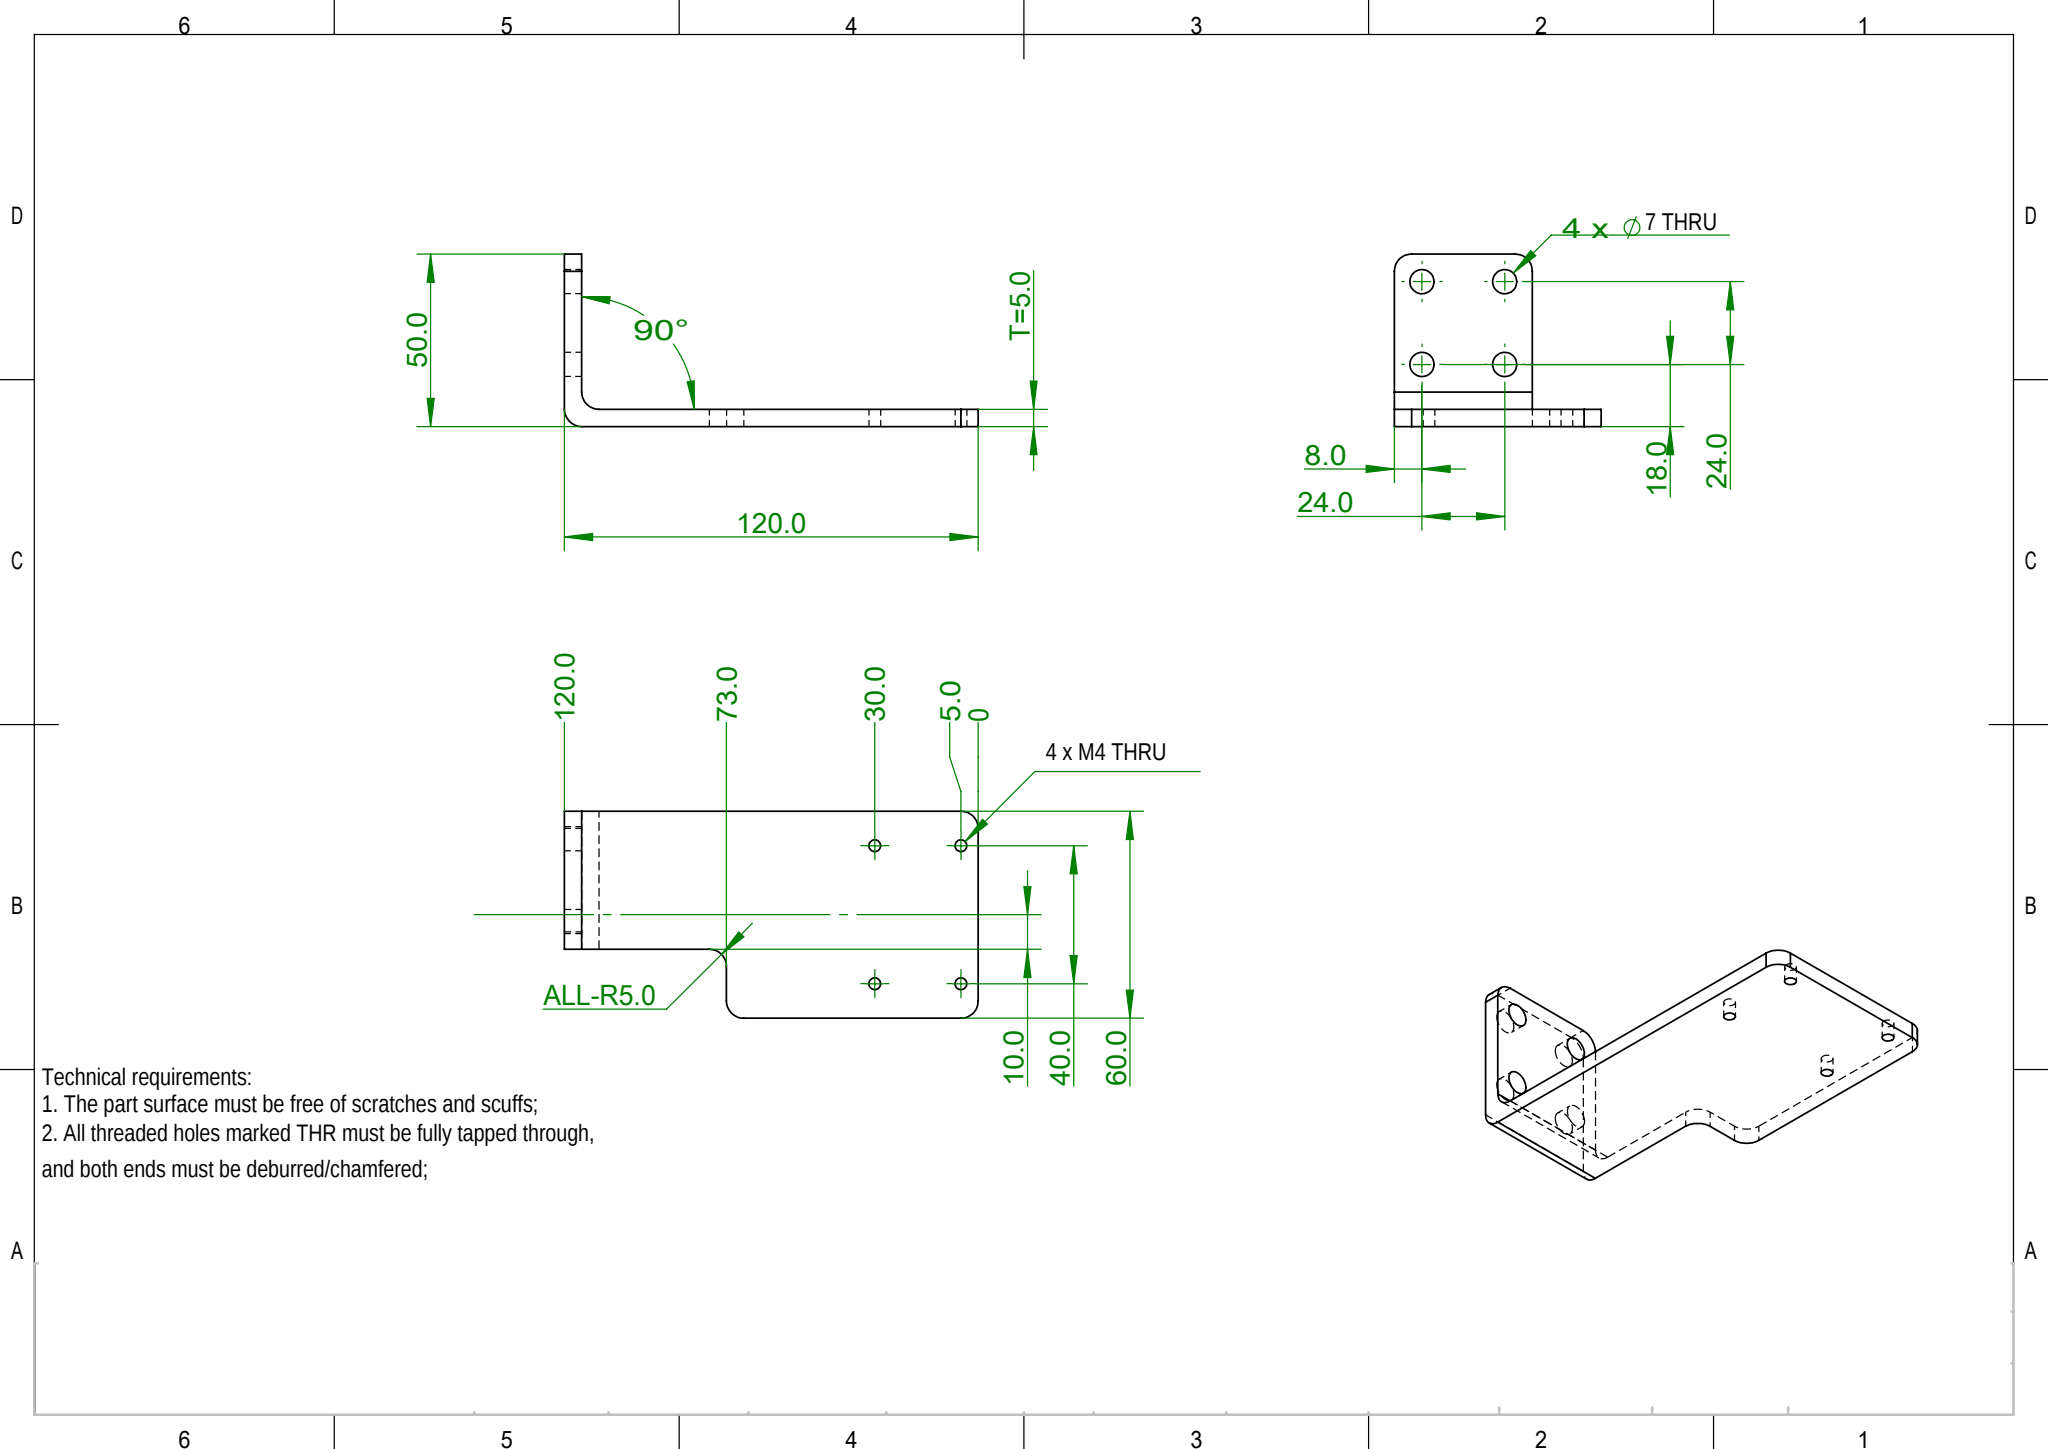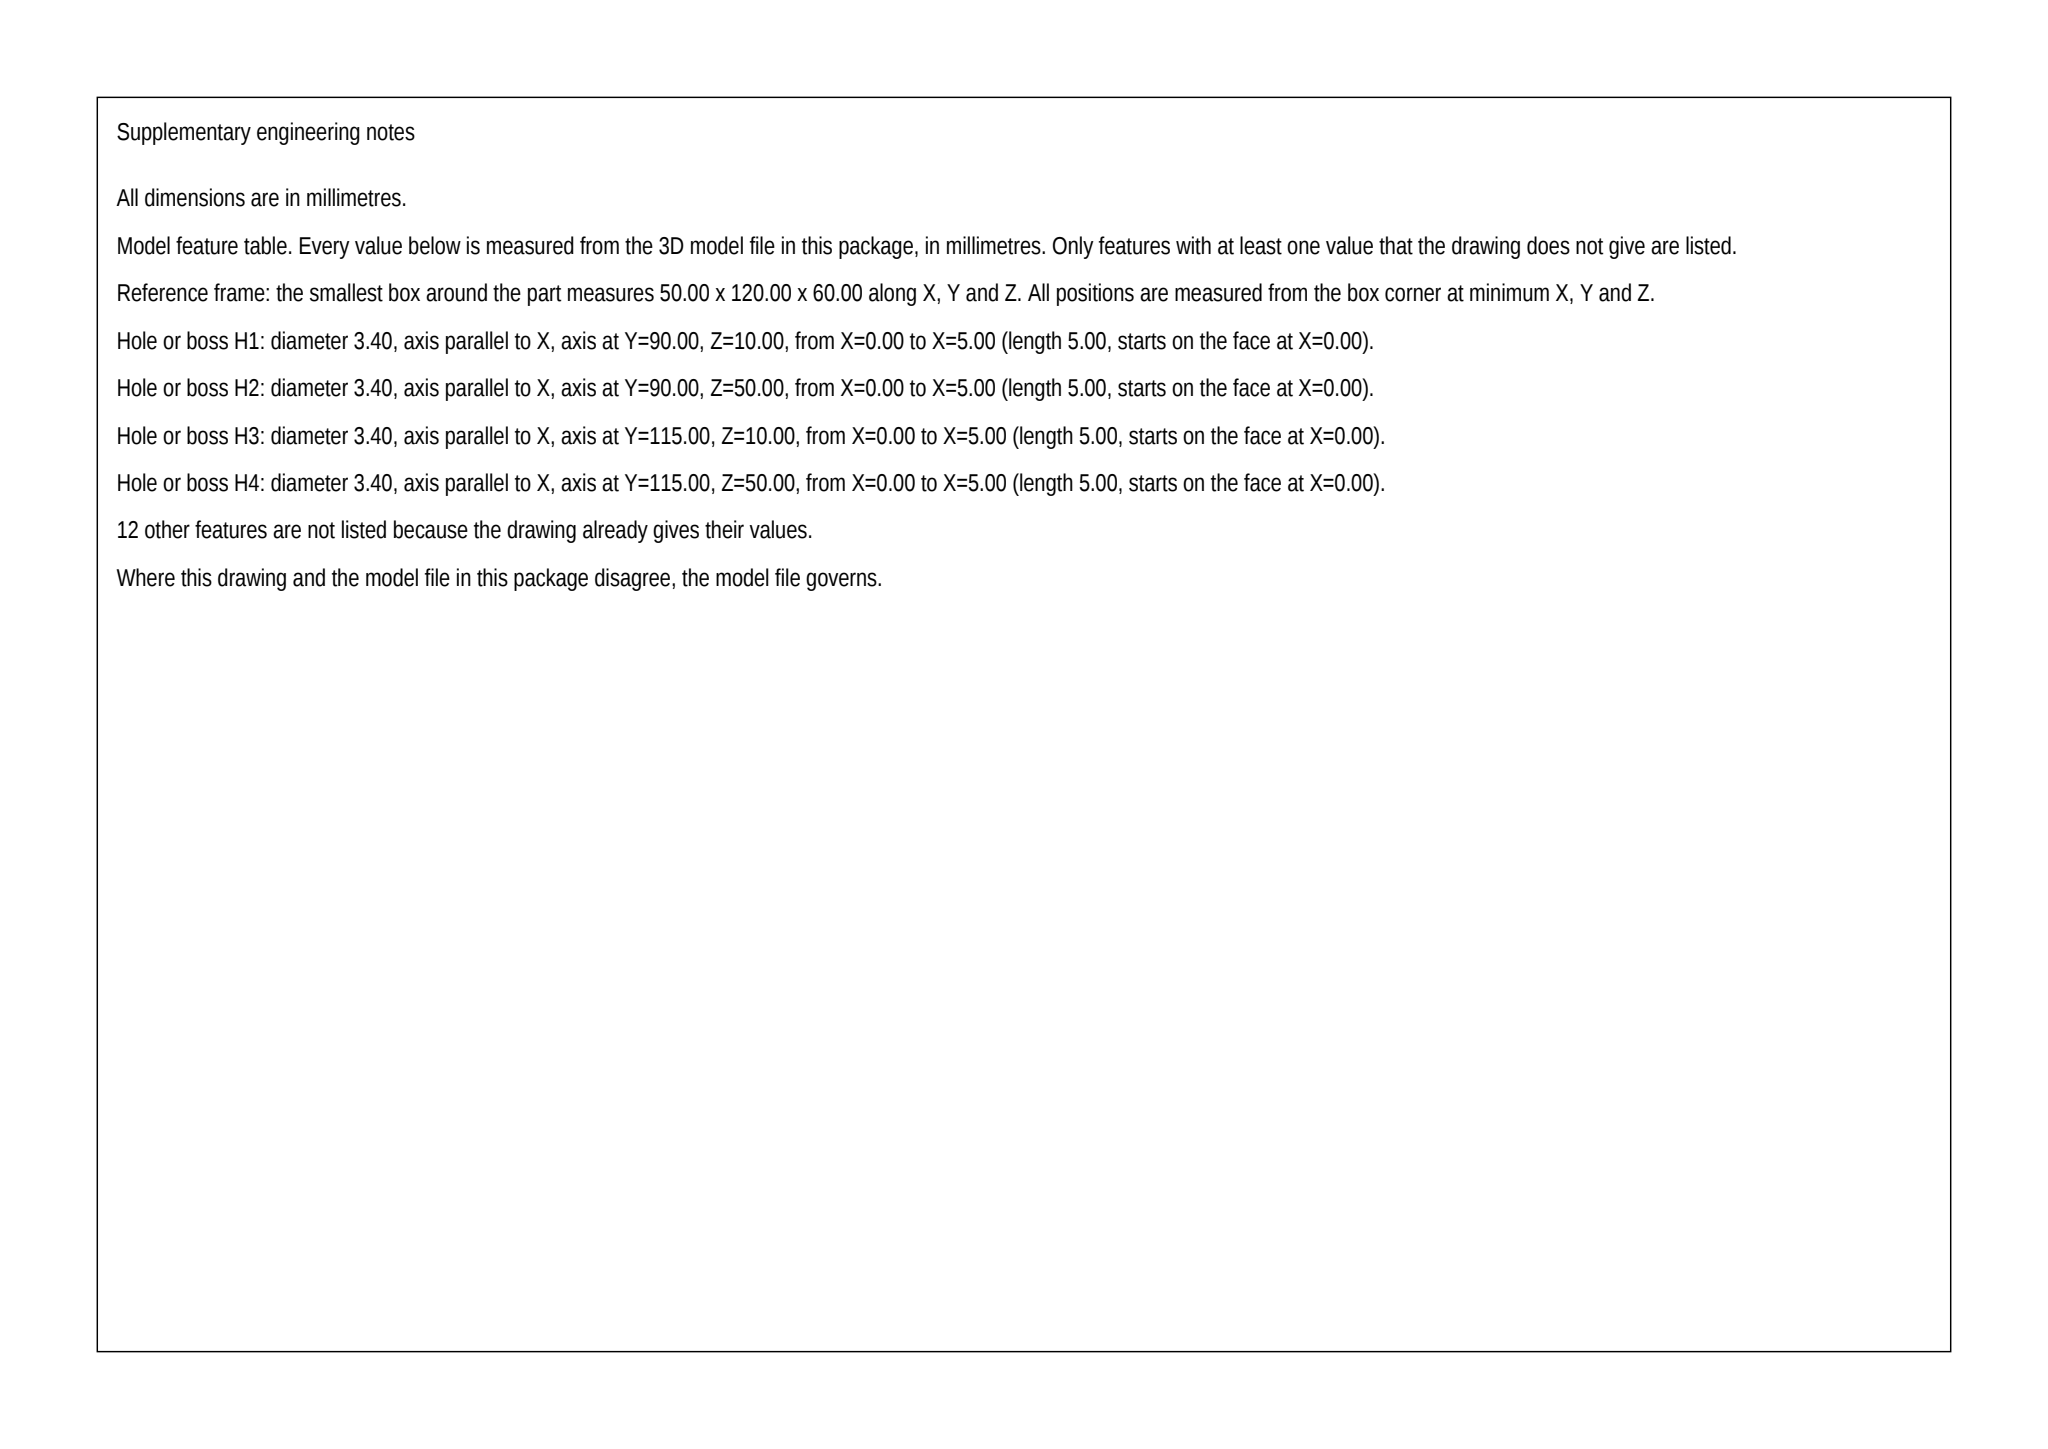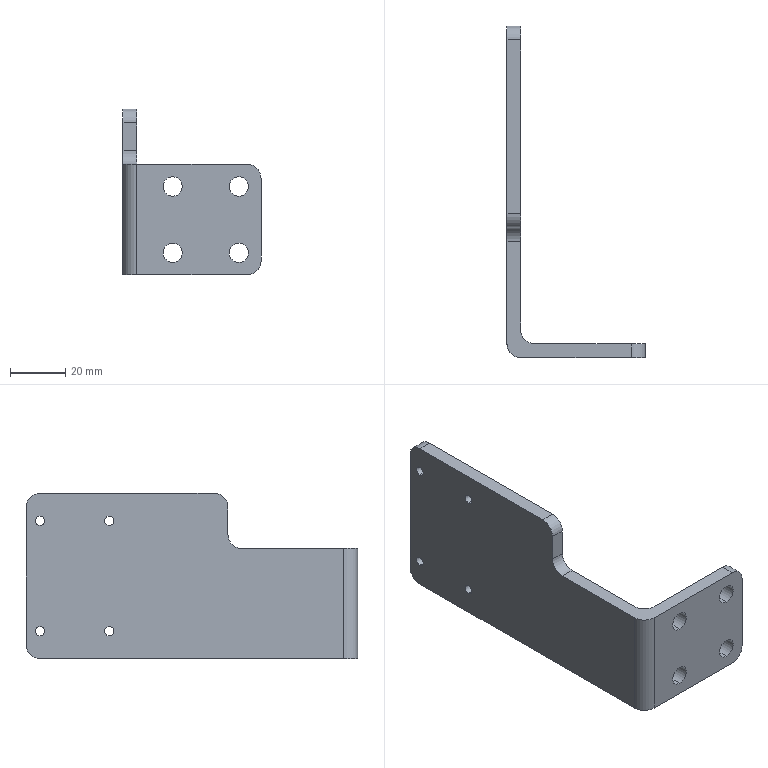Part | SolidWorks | mm | 1 solid | 34 faces | box 50 x 120 x 60 mm | volume 39241 mm3 | cylinder 24 | plane 10 | commonest cylinder face diameters 7 x8 3.4 x8 10 x8